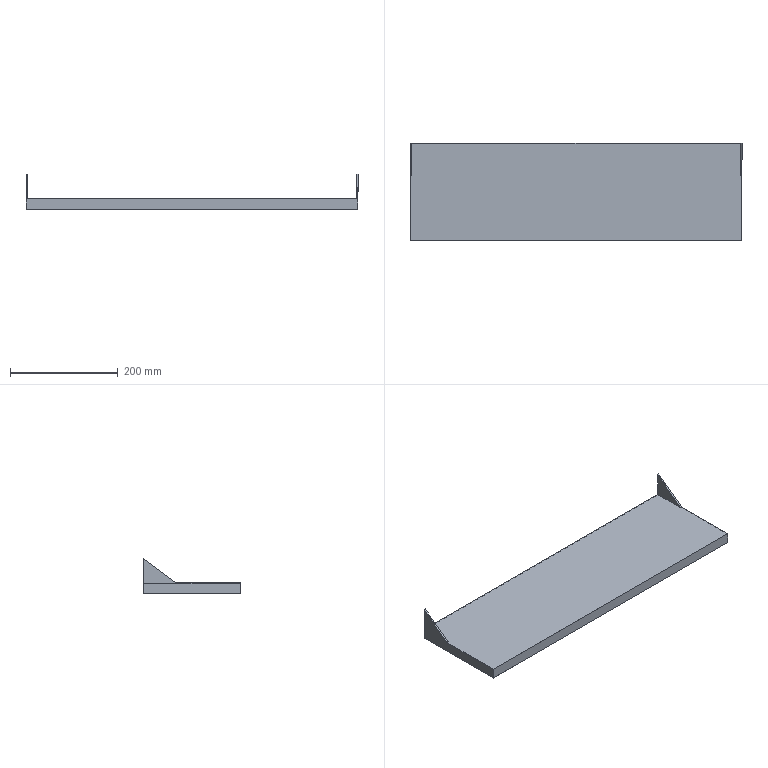Component | SolidWorks | ItemTray-1 | 1 solid | 15 faces | box 616.5 x 181.5 x 65 mm | volume 220065 mm3 | plane 15
STEP:
#1=CARTESIAN_POINT('',(12.343,-8.661,-3.74));
#2=VERTEX_POINT('',#1);
#3=CARTESIAN_POINT('',(12.461,-8.661,-3.74));
#4=VERTEX_POINT('',#3);
#5=CARTESIAN_POINT('',(12.343,-8.661,-3.74));
#6=DIRECTION('',(1.,0.,0.));
#7=VECTOR('',#6,39.37);
#8=LINE('',#5,#7);
#9=EDGE_CURVE('',#2,#4,#8,.T.);
#10=ORIENTED_EDGE('',*,*,#9,.F.);
#11=CARTESIAN_POINT('',(12.343,-6.299,-3.74));
#12=VERTEX_POINT('',#11);
#13=CARTESIAN_POINT('',(12.343,-8.661,-3.74));
#14=DIRECTION('',(0.,-1.,-0.));
#15=VECTOR('',#14,39.37);
#16=LINE('',#13,#15);
#17=EDGE_CURVE('',#12,#2,#16,.T.);
#18=ORIENTED_EDGE('',*,*,#17,.F.);
#19=CARTESIAN_POINT('',(-11.693,-6.299,-3.74));
#20=VERTEX_POINT('',#19);
#21=CARTESIAN_POINT('',(12.431,-6.299,-3.74));
#22=DIRECTION('',(1.,0.,0.));
#23=VECTOR('',#22,39.37);
#24=LINE('',#21,#23);
#25=EDGE_CURVE('',#20,#12,#24,.T.);
#26=ORIENTED_EDGE('',*,*,#25,.F.);
#27=CARTESIAN_POINT('',(-11.693,-8.661,-3.74));
#28=VERTEX_POINT('',#27);
#29=CARTESIAN_POINT('',(-11.693,-8.661,-3.74));
#30=DIRECTION('',(0.,-1.,-0.));
#31=VECTOR('',#30,39.37);
#32=LINE('',#29,#31);
#33=EDGE_CURVE('',#20,#28,#32,.T.);
#34=ORIENTED_EDGE('',*,*,#33,.T.);
#35=CARTESIAN_POINT('',(-11.811,-8.661,-3.74));
#36=VERTEX_POINT('',#35);
#37=CARTESIAN_POINT('',(-11.693,-8.661,-3.74));
#38=DIRECTION('',(-1.,-0.,-0.));
#39=VECTOR('',#38,39.37);
#40=LINE('',#37,#39);
#41=EDGE_CURVE('',#28,#36,#40,.T.);
#42=ORIENTED_EDGE('',*,*,#41,.T.);
#43=CARTESIAN_POINT('',(-11.811,-13.445,-3.74));
#44=VERTEX_POINT('',#43);
#45=CARTESIAN_POINT('',(-11.811,-6.329,-3.74));
#46=DIRECTION('',(-0.,1.,0.));
#47=VECTOR('',#46,39.37);
#48=LINE('',#45,#47);
#49=EDGE_CURVE('',#44,#36,#48,.T.);
#50=ORIENTED_EDGE('',*,*,#49,.F.);
#51=CARTESIAN_POINT('',(12.461,-13.445,-3.74));
#52=VERTEX_POINT('',#51);
#53=CARTESIAN_POINT('',(12.431,-13.445,-3.74));
#54=DIRECTION('',(-1.,-0.,-0.));
#55=VECTOR('',#54,39.37);
#56=LINE('',#53,#55);
#57=EDGE_CURVE('',#52,#44,#56,.T.);
#58=ORIENTED_EDGE('',*,*,#57,.F.);
#59=CARTESIAN_POINT('',(12.461,-6.329,-3.74));
#60=DIRECTION('',(0.,-1.,-0.));
#61=VECTOR('',#60,39.37);
#62=LINE('',#59,#61);
#63=EDGE_CURVE('',#4,#52,#62,.T.);
#64=ORIENTED_EDGE('',*,*,#63,.F.);
#65=EDGE_LOOP('',(#10,#18,#26,#34,#42,#50,#58,#64));
#66=FACE_OUTER_BOUND('',#65,.T.);
#67=CARTESIAN_POINT('',(0.3248,-9.872,-3.74));
#68=DIRECTION('',(0.,0.,-1.));
#69=DIRECTION('',(-1.,-0.,-0.));
#70=AXIS2_PLACEMENT_3D('',#67,#68,#69);
#71=PLANE('',#70);
#72=ADVANCED_FACE('',(#66),#71,.F.);
#73=CARTESIAN_POINT('',(-11.752,-13.386,-3.799));
#74=VERTEX_POINT('',#73);
#75=CARTESIAN_POINT('',(-11.752,-6.358,-3.799));
#76=VERTEX_POINT('',#75);
#77=CARTESIAN_POINT('',(-11.752,-6.329,-3.799));
#78=DIRECTION('',(-0.,1.,0.));
#79=VECTOR('',#78,39.37);
#80=LINE('',#77,#79);
#81=EDGE_CURVE('',#74,#76,#80,.T.);
#82=ORIENTED_EDGE('',*,*,#81,.F.);
#83=CARTESIAN_POINT('',(-11.752,-13.386,-4.528));
#84=VERTEX_POINT('',#83);
#85=CARTESIAN_POINT('',(-11.752,-13.386,-4.469));
#86=DIRECTION('',(-0.,-0.,1.));
#87=VECTOR('',#86,39.37);
#88=LINE('',#85,#87);
#89=EDGE_CURVE('',#84,#74,#88,.T.);
#90=ORIENTED_EDGE('',*,*,#89,.F.);
#91=CARTESIAN_POINT('',(-11.752,-6.358,-4.528));
#92=VERTEX_POINT('',#91);
#93=CARTESIAN_POINT('',(-11.752,-9.872,-4.528));
#94=DIRECTION('',(-0.,1.,0.));
#95=VECTOR('',#94,39.37);
#96=LINE('',#93,#95);
#97=EDGE_CURVE('',#84,#92,#96,.T.);
#98=ORIENTED_EDGE('',*,*,#97,.T.);
#99=CARTESIAN_POINT('',(-11.752,-6.358,-4.469));
#100=DIRECTION('',(-0.,-0.,1.));
#101=VECTOR('',#100,39.37);
#102=LINE('',#99,#101);
#103=EDGE_CURVE('',#92,#76,#102,.T.);
#104=ORIENTED_EDGE('',*,*,#103,.T.);
#105=EDGE_LOOP('',(#82,#90,#98,#104));
#106=FACE_OUTER_BOUND('',#105,.T.);
#107=CARTESIAN_POINT('',(-11.752,-6.329,-4.469));
#108=DIRECTION('',(1.,0.,0.));
#109=DIRECTION('',(0.,0.,-1.));
#110=AXIS2_PLACEMENT_3D('',#107,#108,#109);
#111=PLANE('',#110);
#112=ADVANCED_FACE('',(#106),#111,.T.);
#113=CARTESIAN_POINT('',(12.402,-6.358,-3.799));
#114=VERTEX_POINT('',#113);
#115=CARTESIAN_POINT('',(12.431,-6.358,-3.799));
#116=DIRECTION('',(1.,0.,0.));
#117=VECTOR('',#116,39.37);
#118=LINE('',#115,#117);
#119=EDGE_CURVE('',#76,#114,#118,.T.);
#120=ORIENTED_EDGE('',*,*,#119,.F.);
#121=ORIENTED_EDGE('',*,*,#103,.F.);
#122=CARTESIAN_POINT('',(12.402,-6.358,-4.528));
#123=VERTEX_POINT('',#122);
#124=CARTESIAN_POINT('',(0.3248,-6.358,-4.528));
#125=DIRECTION('',(1.,0.,0.));
#126=VECTOR('',#125,39.37);
#127=LINE('',#124,#126);
#128=EDGE_CURVE('',#92,#123,#127,.T.);
#129=ORIENTED_EDGE('',*,*,#128,.T.);
#130=CARTESIAN_POINT('',(12.402,-6.358,-4.469));
#131=DIRECTION('',(-0.,-0.,1.));
#132=VECTOR('',#131,39.37);
#133=LINE('',#130,#132);
#134=EDGE_CURVE('',#123,#114,#133,.T.);
#135=ORIENTED_EDGE('',*,*,#134,.T.);
#136=EDGE_LOOP('',(#120,#121,#129,#135));
#137=FACE_OUTER_BOUND('',#136,.T.);
#138=CARTESIAN_POINT('',(12.431,-6.358,-4.469));
#139=DIRECTION('',(0.,-1.,-0.));
#140=DIRECTION('',(-0.,-0.,1.));
#141=AXIS2_PLACEMENT_3D('',#138,#139,#140);
#142=PLANE('',#141);
#143=ADVANCED_FACE('',(#137),#142,.T.);
#144=CARTESIAN_POINT('',(12.402,-13.386,-3.799));
#145=VERTEX_POINT('',#144);
#146=CARTESIAN_POINT('',(12.402,-6.329,-3.799));
#147=DIRECTION('',(0.,-1.,-0.));
#148=VECTOR('',#147,39.37);
#149=LINE('',#146,#148);
#150=EDGE_CURVE('',#114,#145,#149,.T.);
#151=ORIENTED_EDGE('',*,*,#150,.F.);
#152=ORIENTED_EDGE('',*,*,#134,.F.);
#153=CARTESIAN_POINT('',(12.402,-13.386,-4.528));
#154=VERTEX_POINT('',#153);
#155=CARTESIAN_POINT('',(12.402,-9.872,-4.528));
#156=DIRECTION('',(0.,-1.,-0.));
#157=VECTOR('',#156,39.37);
#158=LINE('',#155,#157);
#159=EDGE_CURVE('',#123,#154,#158,.T.);
#160=ORIENTED_EDGE('',*,*,#159,.T.);
#161=CARTESIAN_POINT('',(12.402,-13.386,-4.469));
#162=DIRECTION('',(-0.,-0.,1.));
#163=VECTOR('',#162,39.37);
#164=LINE('',#161,#163);
#165=EDGE_CURVE('',#154,#145,#164,.T.);
#166=ORIENTED_EDGE('',*,*,#165,.T.);
#167=EDGE_LOOP('',(#151,#152,#160,#166));
#168=FACE_OUTER_BOUND('',#167,.T.);
#169=CARTESIAN_POINT('',(12.402,-6.329,-4.469));
#170=DIRECTION('',(-1.,-0.,-0.));
#171=DIRECTION('',(-0.,-0.,1.));
#172=AXIS2_PLACEMENT_3D('',#169,#170,#171);
#173=PLANE('',#172);
#174=ADVANCED_FACE('',(#168),#173,.T.);
#175=CARTESIAN_POINT('',(12.431,-13.386,-3.799));
#176=DIRECTION('',(-1.,-0.,-0.));
#177=VECTOR('',#176,39.37);
#178=LINE('',#175,#177);
#179=EDGE_CURVE('',#145,#74,#178,.T.);
#180=ORIENTED_EDGE('',*,*,#179,.F.);
#181=ORIENTED_EDGE('',*,*,#165,.F.);
#182=CARTESIAN_POINT('',(0.3248,-13.386,-4.528));
#183=DIRECTION('',(-1.,-0.,-0.));
#184=VECTOR('',#183,39.37);
#185=LINE('',#182,#184);
#186=EDGE_CURVE('',#154,#84,#185,.T.);
#187=ORIENTED_EDGE('',*,*,#186,.T.);
#188=ORIENTED_EDGE('',*,*,#89,.T.);
#189=EDGE_LOOP('',(#180,#181,#187,#188));
#190=FACE_OUTER_BOUND('',#189,.T.);
#191=CARTESIAN_POINT('',(12.431,-13.386,-4.469));
#192=DIRECTION('',(-0.,1.,0.));
#193=DIRECTION('',(0.,0.,-1.));
#194=AXIS2_PLACEMENT_3D('',#191,#192,#193);
#195=PLANE('',#194);
#196=ADVANCED_FACE('',(#190),#195,.T.);
#197=ORIENTED_EDGE('',*,*,#81,.T.);
#198=ORIENTED_EDGE('',*,*,#119,.T.);
#199=ORIENTED_EDGE('',*,*,#150,.T.);
#200=ORIENTED_EDGE('',*,*,#179,.T.);
#201=EDGE_LOOP('',(#197,#198,#199,#200));
#202=FACE_OUTER_BOUND('',#201,.T.);
#203=CARTESIAN_POINT('',(0.3248,-9.872,-3.799));
#204=DIRECTION('',(0.,0.,-1.));
#205=DIRECTION('',(-1.,-0.,-0.));
#206=AXIS2_PLACEMENT_3D('',#203,#204,#205);
#207=PLANE('',#206);
#208=ADVANCED_FACE('',(#202),#207,.T.);
#209=ORIENTED_EDGE('',*,*,#49,.T.);
#210=CARTESIAN_POINT('',(-11.811,-6.299,-1.969));
#211=VERTEX_POINT('',#210);
#212=CARTESIAN_POINT('',(-11.811,-6.299,-1.969));
#213=DIRECTION('',(-0.,0.8,0.6));
#214=VECTOR('',#213,39.37);
#215=LINE('',#212,#214);
#216=EDGE_CURVE('',#36,#211,#215,.T.);
#217=ORIENTED_EDGE('',*,*,#216,.T.);
#218=CARTESIAN_POINT('',(-11.811,-6.299,-4.528));
#219=VERTEX_POINT('',#218);
#220=CARTESIAN_POINT('',(-11.811,-6.299,-4.528));
#221=DIRECTION('',(-0.,-0.,1.));
#222=VECTOR('',#221,39.37);
#223=LINE('',#220,#222);
#224=EDGE_CURVE('',#219,#211,#223,.T.);
#225=ORIENTED_EDGE('',*,*,#224,.F.);
#226=CARTESIAN_POINT('',(-11.811,-13.445,-4.528));
#227=VERTEX_POINT('',#226);
#228=CARTESIAN_POINT('',(-11.811,-6.329,-4.528));
#229=DIRECTION('',(-0.,1.,0.));
#230=VECTOR('',#229,39.37);
#231=LINE('',#228,#230);
#232=EDGE_CURVE('',#227,#219,#231,.T.);
#233=ORIENTED_EDGE('',*,*,#232,.F.);
#234=CARTESIAN_POINT('',(-11.811,-13.445,-4.528));
#235=DIRECTION('',(-0.,-0.,1.));
#236=VECTOR('',#235,39.37);
#237=LINE('',#234,#236);
#238=EDGE_CURVE('',#227,#44,#237,.T.);
#239=ORIENTED_EDGE('',*,*,#238,.T.);
#240=EDGE_LOOP('',(#209,#217,#225,#233,#239));
#241=FACE_OUTER_BOUND('',#240,.T.);
#242=CARTESIAN_POINT('',(-11.811,-6.329,-4.528));
#243=DIRECTION('',(1.,0.,0.));
#244=DIRECTION('',(0.,0.,-1.));
#245=AXIS2_PLACEMENT_3D('',#242,#243,#244);
#246=PLANE('',#245);
#247=ADVANCED_FACE('',(#241),#246,.F.);
#248=ORIENTED_EDGE('',*,*,#224,.T.);
#249=CARTESIAN_POINT('',(-11.693,-6.299,-1.969));
#250=VERTEX_POINT('',#249);
#251=CARTESIAN_POINT('',(-11.693,-6.299,-1.969));
#252=DIRECTION('',(-1.,-0.,-0.));
#253=VECTOR('',#252,39.37);
#254=LINE('',#251,#253);
#255=EDGE_CURVE('',#250,#211,#254,.T.);
#256=ORIENTED_EDGE('',*,*,#255,.F.);
#257=CARTESIAN_POINT('',(-11.693,-6.299,-3.74));
#258=DIRECTION('',(0.,0.,-1.));
#259=VECTOR('',#258,39.37);
#260=LINE('',#257,#259);
#261=EDGE_CURVE('',#250,#20,#260,.T.);
#262=ORIENTED_EDGE('',*,*,#261,.T.);
#263=ORIENTED_EDGE('',*,*,#25,.T.);
#264=CARTESIAN_POINT('',(12.343,-6.299,-1.969));
#265=VERTEX_POINT('',#264);
#266=CARTESIAN_POINT('',(12.343,-6.299,-3.74));
#267=DIRECTION('',(0.,0.,-1.));
#268=VECTOR('',#267,39.37);
#269=LINE('',#266,#268);
#270=EDGE_CURVE('',#265,#12,#269,.T.);
#271=ORIENTED_EDGE('',*,*,#270,.F.);
#272=CARTESIAN_POINT('',(12.461,-6.299,-1.969));
#273=VERTEX_POINT('',#272);
#274=CARTESIAN_POINT('',(12.343,-6.299,-1.969));
#275=DIRECTION('',(1.,0.,0.));
#276=VECTOR('',#275,39.37);
#277=LINE('',#274,#276);
#278=EDGE_CURVE('',#265,#273,#277,.T.);
#279=ORIENTED_EDGE('',*,*,#278,.T.);
#280=CARTESIAN_POINT('',(12.461,-6.299,-4.528));
#281=VERTEX_POINT('',#280);
#282=CARTESIAN_POINT('',(12.461,-6.299,-4.528));
#283=DIRECTION('',(-0.,-0.,1.));
#284=VECTOR('',#283,39.37);
#285=LINE('',#282,#284);
#286=EDGE_CURVE('',#281,#273,#285,.T.);
#287=ORIENTED_EDGE('',*,*,#286,.F.);
#288=CARTESIAN_POINT('',(12.431,-6.299,-4.528));
#289=DIRECTION('',(1.,0.,0.));
#290=VECTOR('',#289,39.37);
#291=LINE('',#288,#290);
#292=EDGE_CURVE('',#219,#281,#291,.T.);
#293=ORIENTED_EDGE('',*,*,#292,.F.);
#294=EDGE_LOOP('',(#248,#256,#262,#263,#271,#279,#287,#293));
#295=FACE_OUTER_BOUND('',#294,.T.);
#296=CARTESIAN_POINT('',(12.431,-6.299,-4.528));
#297=DIRECTION('',(0.,-1.,-0.));
#298=DIRECTION('',(-0.,-0.,1.));
#299=AXIS2_PLACEMENT_3D('',#296,#297,#298);
#300=PLANE('',#299);
#301=ADVANCED_FACE('',(#295),#300,.F.);
#302=ORIENTED_EDGE('',*,*,#286,.T.);
#303=CARTESIAN_POINT('',(12.461,-6.299,-1.969));
#304=DIRECTION('',(-0.,0.8,0.6));
#305=VECTOR('',#304,39.37);
#306=LINE('',#303,#305);
#307=EDGE_CURVE('',#4,#273,#306,.T.);
#308=ORIENTED_EDGE('',*,*,#307,.F.);
#309=ORIENTED_EDGE('',*,*,#63,.T.);
#310=CARTESIAN_POINT('',(12.461,-13.445,-4.528));
#311=VERTEX_POINT('',#310);
#312=CARTESIAN_POINT('',(12.461,-13.445,-4.528));
#313=DIRECTION('',(-0.,-0.,1.));
#314=VECTOR('',#313,39.37);
#315=LINE('',#312,#314);
#316=EDGE_CURVE('',#311,#52,#315,.T.);
#317=ORIENTED_EDGE('',*,*,#316,.F.);
#318=CARTESIAN_POINT('',(12.461,-6.329,-4.528));
#319=DIRECTION('',(0.,-1.,-0.));
#320=VECTOR('',#319,39.37);
#321=LINE('',#318,#320);
#322=EDGE_CURVE('',#281,#311,#321,.T.);
#323=ORIENTED_EDGE('',*,*,#322,.F.);
#324=EDGE_LOOP('',(#302,#308,#309,#317,#323));
#325=FACE_OUTER_BOUND('',#324,.T.);
#326=CARTESIAN_POINT('',(12.461,-6.329,-4.528));
#327=DIRECTION('',(-1.,-0.,-0.));
#328=DIRECTION('',(-0.,-0.,1.));
#329=AXIS2_PLACEMENT_3D('',#326,#327,#328);
#330=PLANE('',#329);
#331=ADVANCED_FACE('',(#325),#330,.F.);
#332=ORIENTED_EDGE('',*,*,#57,.T.);
#333=ORIENTED_EDGE('',*,*,#238,.F.);
#334=CARTESIAN_POINT('',(12.431,-13.445,-4.528));
#335=DIRECTION('',(-1.,-0.,-0.));
#336=VECTOR('',#335,39.37);
#337=LINE('',#334,#336);
#338=EDGE_CURVE('',#311,#227,#337,.T.);
#339=ORIENTED_EDGE('',*,*,#338,.F.);
#340=ORIENTED_EDGE('',*,*,#316,.T.);
#341=EDGE_LOOP('',(#332,#333,#339,#340));
#342=FACE_OUTER_BOUND('',#341,.T.);
#343=CARTESIAN_POINT('',(12.431,-13.445,-4.528));
#344=DIRECTION('',(-0.,1.,0.));
#345=DIRECTION('',(0.,0.,-1.));
#346=AXIS2_PLACEMENT_3D('',#343,#344,#345);
#347=PLANE('',#346);
#348=ADVANCED_FACE('',(#342),#347,.F.);
#349=ORIENTED_EDGE('',*,*,#128,.F.);
#350=ORIENTED_EDGE('',*,*,#97,.F.);
#351=ORIENTED_EDGE('',*,*,#186,.F.);
#352=ORIENTED_EDGE('',*,*,#159,.F.);
#353=EDGE_LOOP('',(#349,#350,#351,#352));
#354=FACE_BOUND('',#353,.T.);
#355=ORIENTED_EDGE('',*,*,#232,.T.);
#356=ORIENTED_EDGE('',*,*,#292,.T.);
#357=ORIENTED_EDGE('',*,*,#322,.T.);
#358=ORIENTED_EDGE('',*,*,#338,.T.);
#359=EDGE_LOOP('',(#355,#356,#357,#358));
#360=FACE_OUTER_BOUND('',#359,.T.);
#361=CARTESIAN_POINT('',(0.3248,-9.872,-4.528));
#362=DIRECTION('',(0.,0.,-1.));
#363=DIRECTION('',(-1.,-0.,-0.));
#364=AXIS2_PLACEMENT_3D('',#361,#362,#363);
#365=PLANE('',#364);
#366=ADVANCED_FACE('',(#354,#360),#365,.T.);
#367=ORIENTED_EDGE('',*,*,#216,.F.);
#368=ORIENTED_EDGE('',*,*,#41,.F.);
#369=CARTESIAN_POINT('',(-11.693,-6.299,-1.969));
#370=DIRECTION('',(-0.,0.8,0.6));
#371=VECTOR('',#370,39.37);
#372=LINE('',#369,#371);
#373=EDGE_CURVE('',#28,#250,#372,.T.);
#374=ORIENTED_EDGE('',*,*,#373,.T.);
#375=ORIENTED_EDGE('',*,*,#255,.T.);
#376=EDGE_LOOP('',(#367,#368,#374,#375));
#377=FACE_OUTER_BOUND('',#376,.T.);
#378=CARTESIAN_POINT('',(-11.693,-6.299,-1.969));
#379=DIRECTION('',(0.,-0.6,0.8));
#380=DIRECTION('',(-0.,0.8,0.6));
#381=AXIS2_PLACEMENT_3D('',#378,#379,#380);
#382=PLANE('',#381);
#383=ADVANCED_FACE('',(#377),#382,.T.);
#384=ORIENTED_EDGE('',*,*,#33,.F.);
#385=ORIENTED_EDGE('',*,*,#261,.F.);
#386=ORIENTED_EDGE('',*,*,#373,.F.);
#387=EDGE_LOOP('',(#384,#385,#386));
#388=FACE_OUTER_BOUND('',#387,.T.);
#389=CARTESIAN_POINT('',(-11.693,-9.872,-3.74));
#390=DIRECTION('',(1.,0.,0.));
#391=DIRECTION('',(0.,0.,-1.));
#392=AXIS2_PLACEMENT_3D('',#389,#390,#391);
#393=PLANE('',#392);
#394=ADVANCED_FACE('',(#388),#393,.T.);
#395=ORIENTED_EDGE('',*,*,#307,.T.);
#396=ORIENTED_EDGE('',*,*,#278,.F.);
#397=CARTESIAN_POINT('',(12.343,-6.299,-1.969));
#398=DIRECTION('',(-0.,0.8,0.6));
#399=VECTOR('',#398,39.37);
#400=LINE('',#397,#399);
#401=EDGE_CURVE('',#2,#265,#400,.T.);
#402=ORIENTED_EDGE('',*,*,#401,.F.);
#403=ORIENTED_EDGE('',*,*,#9,.T.);
#404=EDGE_LOOP('',(#395,#396,#402,#403));
#405=FACE_OUTER_BOUND('',#404,.T.);
#406=CARTESIAN_POINT('',(12.343,-6.299,-1.969));
#407=DIRECTION('',(-0.,0.6,-0.8));
#408=DIRECTION('',(0.,-0.8,-0.6));
#409=AXIS2_PLACEMENT_3D('',#406,#407,#408);
#410=PLANE('',#409);
#411=ADVANCED_FACE('',(#405),#410,.F.);
#412=ORIENTED_EDGE('',*,*,#17,.T.);
#413=ORIENTED_EDGE('',*,*,#401,.T.);
#414=ORIENTED_EDGE('',*,*,#270,.T.);
#415=EDGE_LOOP('',(#412,#413,#414));
#416=FACE_OUTER_BOUND('',#415,.T.);
#417=CARTESIAN_POINT('',(12.343,-9.872,-3.74));
#418=DIRECTION('',(-1.,-0.,-0.));
#419=DIRECTION('',(0.,0.,-1.));
#420=AXIS2_PLACEMENT_3D('',#417,#418,#419);
#421=PLANE('',#420);
#422=ADVANCED_FACE('',(#416),#421,.T.);
#423=CLOSED_SHELL('',(#72,#112,#143,#174,#196,#208,#247,#301,#331,#348,#366,#383,#394,#411,#422));
#424=MANIFOLD_SOLID_BREP('',#423);
#425=CARTESIAN_POINT('',(0.,0.,0.));
#426=DIRECTION('',(0.,0.,1.));
#427=DIRECTION('',(1.,0.,0.));
#428=AXIS2_PLACEMENT_3D('',#425,#426,#427);
#429=(LENGTH_UNIT()NAMED_UNIT(*)SI_UNIT($,.METRE.));
#430=LENGTH_MEASURE_WITH_UNIT(LENGTH_MEASURE(0.0254),#429);
#431=DIMENSIONAL_EXPONENTS(1.,0.,0.,0.,0.,0.,0.);
#432=(CONVERSION_BASED_UNIT('',#430)LENGTH_UNIT()NAMED_UNIT(#431));
#433=UNCERTAINTY_MEASURE_WITH_UNIT(LENGTH_MEASURE(0.00001),#432,'','');
#434=(NAMED_UNIT(*)PLANE_ANGLE_UNIT()SI_UNIT($,.RADIAN.));
#435=(NAMED_UNIT(*)SI_UNIT($,.STERADIAN.)SOLID_ANGLE_UNIT());
#436=(GEOMETRIC_REPRESENTATION_CONTEXT(3)GLOBAL_UNCERTAINTY_ASSIGNED_CONTEXT((#433))GLOBAL_UNIT_ASSIGNED_CONTEXT((#432,#434,#435))REPRESENTATION_CONTEXT('',''));
#437=ADVANCED_BREP_SHAPE_REPRESENTATION('',(#424,#428),#436);
#438=COLOUR_RGB('',0.7922,0.8196,0.9333);
#439=FILL_AREA_STYLE_COLOUR('',#438);
#440=FILL_AREA_STYLE('',(#439));
#441=SURFACE_STYLE_FILL_AREA(#440);
#442=SURFACE_SIDE_STYLE('',(#441));
#443=SURFACE_STYLE_USAGE(.BOTH.,#442);
#444=PRESENTATION_STYLE_ASSIGNMENT((#443));
#445=STYLED_ITEM('',(#444),#424);
#446=(LENGTH_UNIT()NAMED_UNIT(*)SI_UNIT($,.METRE.));
#447=LENGTH_MEASURE_WITH_UNIT(LENGTH_MEASURE(0.0254),#446);
#448=DIMENSIONAL_EXPONENTS(1.,0.,0.,0.,0.,0.,0.);
#449=(CONVERSION_BASED_UNIT('',#447)LENGTH_UNIT()NAMED_UNIT(#448));
#450=UNCERTAINTY_MEASURE_WITH_UNIT(LENGTH_MEASURE(0.00001),#449,'','');
#451=(NAMED_UNIT(*)PLANE_ANGLE_UNIT()SI_UNIT($,.RADIAN.));
#452=(NAMED_UNIT(*)SI_UNIT($,.STERADIAN.)SOLID_ANGLE_UNIT());
#453=(GEOMETRIC_REPRESENTATION_CONTEXT(3)GLOBAL_UNCERTAINTY_ASSIGNED_CONTEXT((#450))GLOBAL_UNIT_ASSIGNED_CONTEXT((#449,#451,#452))REPRESENTATION_CONTEXT('',''));
#454=MECHANICAL_DESIGN_GEOMETRIC_PRESENTATION_REPRESENTATION('',(#445),#453);
#455=PRESENTATION_LAYER_ASSIGNMENT('','',(#445));